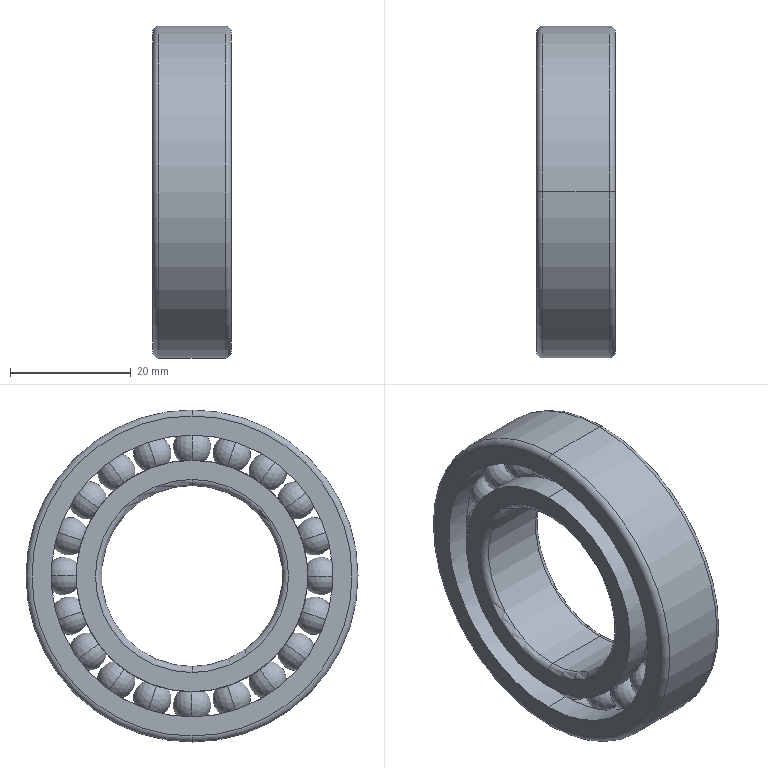Component | SolidWorks | LowerSideBeltXG-XG1-1_GB6006BearingXG-XG1-1 | 1 solid | 124 faces | box 13 x 55 x 55 mm | volume 16022 mm3 | torus 68 | sphere 40 | cylinder 12 | plane 4 | commonest cylinder face diameters 46.667 x4 38.333 x4 55 x2 30 x2
build123d program:
from build123d import *

# Parameters (mm, degrees)
CIRCULAR_PATTERN1_COUNT = 20
FILLET1_R               = 1


with BuildPart() as part:
    # Sketch1 → Revolve1 (revolve)
    with BuildSketch(Plane.XY):
        with BuildLine():
            Line((-3.125, 21.25), (3.125, 21.25))
            ThreePointArc((3.125, 21.25), (0, 24.375), (-3.125, 21.25))
        make_face()
    revolve1 = revolve(axis=Axis((-4.597, 21.25, 0), (1, 0, 0)))

    # Sketch2 → Revolve2 (revolve)
    with BuildSketch(Plane.XY, mode=Mode.PRIVATE) as revolve2_sk:
        with BuildLine():
            Line((-6.5, 19.167), (-6.5, 15))
            Line((-6.5, 15), (6.5, 15))
            Line((6.5, 15), (6.5, 19.167))
            Line((6.5, 19.167), (2.316, 19.167))
            ThreePointArc((2.316, 19.167), (0, 18.135), (-2.316, 19.167))
            Line((-2.316, 19.167), (-6.5, 19.167))
        make_face()
    revolve(revolve2_sk.sketch.rotate(Axis((-6.971, 0, 0), (1, 0, 0)), 90), axis=Axis((-6.971, 0, 0), (1, 0, 0)))

    # Sketch3 → Revolve3 (revolve)
    with BuildSketch(Plane.XY, mode=Mode.PRIVATE) as revolve3_sk:
        with BuildLine():
            Line((-6.5, 27.5), (6.5, 27.5))
            Line((6.5, 27.5), (6.5, 23.333))
            Line((6.5, 23.333), (2.316, 23.333))
            ThreePointArc((2.316, 23.333), (0, 24.365), (-2.316, 23.333))
            Line((-2.316, 23.333), (-6.5, 23.333))
            Line((-6.5, 23.333), (-6.5, 27.5))
        make_face()
    revolve(revolve3_sk.sketch.rotate(Axis((-8.711, 0, 0), (1, 0, 0)), 90), axis=Axis((-8.711, 0, 0), (1, 0, 0)))

    # Circular-Pattern1: Revolve1 ×20 about axis
    circular_pattern1_axis = Axis((0, 0, 0), (1, 0, 0))
    for i in range(1, CIRCULAR_PATTERN1_COUNT):
        add(revolve1.rotate(circular_pattern1_axis, i * 360 / CIRCULAR_PATTERN1_COUNT))

    # Fillet1
    fillet1_edges = [part.edges().sort_by_distance(p)[0] for p in [
        (-6.5, 0, -27.5),
        (6.5, 0, -27.5),
        (-6.5, 0, -15),
        (6.5, 0, -15),
    ]]
    fillet(fillet1_edges, radius=FILLET1_R)


solid = part.part

# Placed as in the assembly
solid = solid.moved(Location((-309.72, 625, 114), (0, 0, 0)))